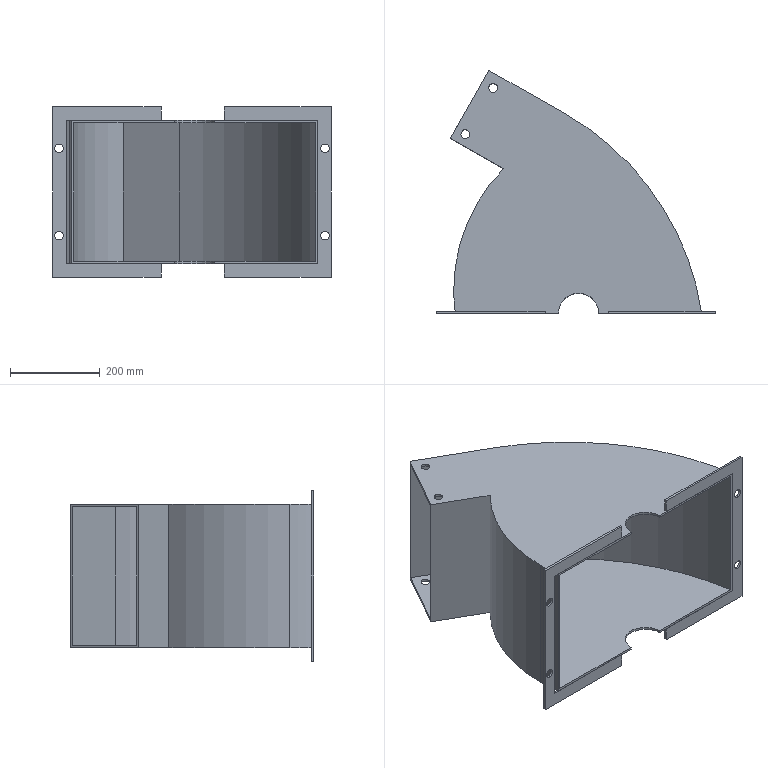Component | SolidWorks | UpperHousing1-1 | 3 solids | 55 faces | volume 4119464 mm3 | plane 31 | cylinder 24 | commonest cylinder face diameters 19.263 x8 19.801 x8 767.637 x2 757.637 x2 90 x2 1236.316 x1 1226.316 x1